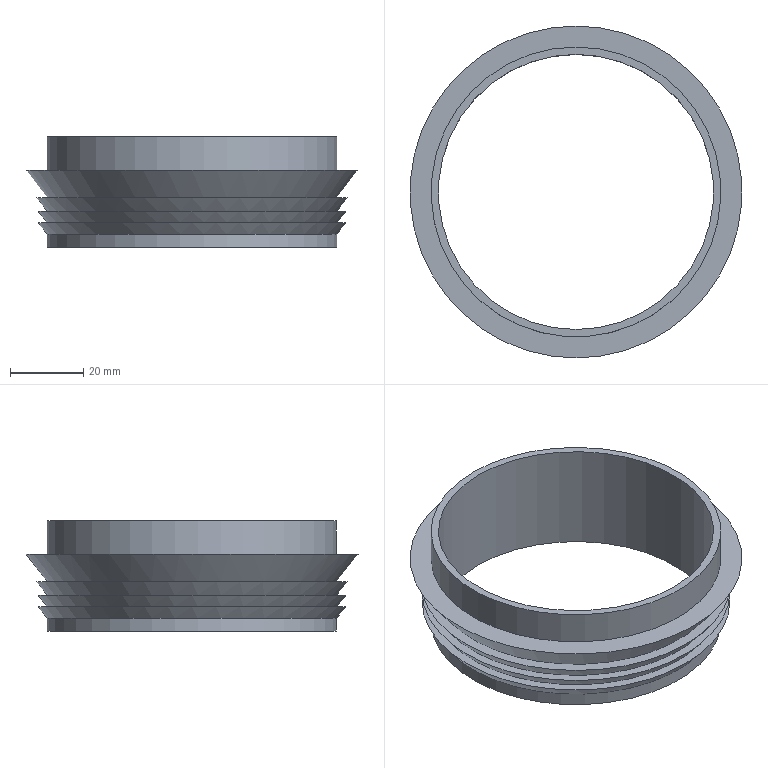Component | NX | CA6140-ZHUZHOU-MIFENGQUAN | 1 solid | 13 faces | box 90.5 x 90.5 x 30 mm | volume 23347 mm3 | plane 6 | cone 4 | cylinder 3 | commonest cylinder face diameters 79 x2 75 x1
STEP:
#1=CARTESIAN_POINT('',(0.,0.,0.));
#2=DIRECTION('',(0.,0.,1.));
#3=DIRECTION('',(1.,0.,0.));
#4=AXIS2_PLACEMENT_3D('',#1,#2,#3);
#5=CARTESIAN_POINT('',(-0.,39.5,-629.951));
#6=VERTEX_POINT('',#5);
#7=CARTESIAN_POINT('',(-0.,0.,-629.951));
#8=DIRECTION('',(0.,0.,-1.));
#9=DIRECTION('',(0.,1.,0.));
#10=AXIS2_PLACEMENT_3D('',#7,#8,#9);
#11=CIRCLE('',#10,39.5);
#12=CARTESIAN_POINT('',(-0.,0.,-629.951));
#13=DIRECTION('',(0.,0.,-1.));
#14=DIRECTION('',(0.,1.,0.));
#15=AXIS2_PLACEMENT_3D('',#12,#13,#14);
#16=CYLINDRICAL_SURFACE('',#15,39.5);
#17=CARTESIAN_POINT('',(0.,0.));
#18=DIRECTION('',(1.,0.));
#19=VECTOR('',#18,1.);
#20=LINE('',#17,#19);
#21=(GEOMETRIC_REPRESENTATION_CONTEXT(2)PARAMETRIC_REPRESENTATION_CONTEXT()REPRESENTATION_CONTEXT('',''));
#22=DEFINITIONAL_REPRESENTATION('',(#20),#21);
#23=PCURVE('',#16,#22);
#24=CARTESIAN_POINT('',(-0.,-39.5,-629.951));
#25=DIRECTION('',(0.,0.,1.));
#26=DIRECTION('',(0.,-1.,0.));
#27=AXIS2_PLACEMENT_3D('',#24,#25,#26);
#28=PLANE('',#27);
#29=CARTESIAN_POINT('',(-79.,0.));
#30=CARTESIAN_POINT('',(-79.,68.416));
#31=CARTESIAN_POINT('',(-19.75,34.208));
#32=CARTESIAN_POINT('',(39.5,0.));
#33=CARTESIAN_POINT('',(-19.75,-34.208));
#34=CARTESIAN_POINT('',(-79.,-68.416));
#35=CARTESIAN_POINT('',(-79.,0.));
#36=(BOUNDED_CURVE()B_SPLINE_CURVE(2,(#29,#30,#31,#32,#33,#34,#35),.UNSPECIFIED.,.T.,.F.)B_SPLINE_CURVE_WITH_KNOTS((1,2,2,2,2,1),(-2.094,0.,2.094,4.189,6.283,8.378),.UNSPECIFIED.)CURVE()GEOMETRIC_REPRESENTATION_ITEM()RATIONAL_B_SPLINE_CURVE((1.,0.5,1.,0.5,1.,0.5,1.))REPRESENTATION_ITEM(''));
#37=(GEOMETRIC_REPRESENTATION_CONTEXT(2)PARAMETRIC_REPRESENTATION_CONTEXT()REPRESENTATION_CONTEXT('',''));
#38=DEFINITIONAL_REPRESENTATION('',(#36),#37);
#39=PCURVE('',#28,#38);
#40=SURFACE_CURVE('',#11,(#23,#39),.PCURVE_S1.);
#41=EDGE_CURVE('',#6,#6,#40,.T.);
#42=ORIENTED_EDGE('',*,*,#41,.F.);
#43=CARTESIAN_POINT('',(-0.,39.5,-626.451));
#44=VERTEX_POINT('',#43);
#45=CARTESIAN_POINT('',(-0.,39.5,-626.451));
#46=CARTESIAN_POINT('',(-0.,39.5,-629.951));
#47=B_SPLINE_CURVE_WITH_KNOTS('',1,(#45,#46),.UNSPECIFIED.,.F.,.F.,(2,2),(-3.5,0.),.PIECEWISE_BEZIER_KNOTS.);
#48=CARTESIAN_POINT('',(0.,0.));
#49=DIRECTION('',(0.,1.));
#50=VECTOR('',#49,1.);
#51=LINE('',#48,#50);
#52=(GEOMETRIC_REPRESENTATION_CONTEXT(2)PARAMETRIC_REPRESENTATION_CONTEXT()REPRESENTATION_CONTEXT('',''));
#53=DEFINITIONAL_REPRESENTATION('',(#51),#52);
#54=PCURVE('',#16,#53);
#55=CARTESIAN_POINT('',(6.283,0.));
#56=DIRECTION('',(0.,1.));
#57=VECTOR('',#56,1.);
#58=LINE('',#55,#57);
#59=(GEOMETRIC_REPRESENTATION_CONTEXT(2)PARAMETRIC_REPRESENTATION_CONTEXT()REPRESENTATION_CONTEXT('',''));
#60=DEFINITIONAL_REPRESENTATION('',(#58),#59);
#61=PCURVE('',#16,#60);
#62=SEAM_CURVE('',#47,(#54,#61),.PCURVE_S1.);
#63=EDGE_CURVE('',#44,#6,#62,.T.);
#64=ORIENTED_EDGE('',*,*,#63,.F.);
#65=CARTESIAN_POINT('',(-0.,0.,-626.451));
#66=DIRECTION('',(0.,0.,-1.));
#67=DIRECTION('',(0.,1.,0.));
#68=AXIS2_PLACEMENT_3D('',#65,#66,#67);
#69=CIRCLE('',#68,39.5);
#70=CARTESIAN_POINT('',(0.,-3.5));
#71=DIRECTION('',(1.,0.));
#72=VECTOR('',#71,1.);
#73=LINE('',#70,#72);
#74=(GEOMETRIC_REPRESENTATION_CONTEXT(2)PARAMETRIC_REPRESENTATION_CONTEXT()REPRESENTATION_CONTEXT('',''));
#75=DEFINITIONAL_REPRESENTATION('',(#73),#74);
#76=PCURVE('',#16,#75);
#77=CARTESIAN_POINT('',(-0.,0.,-623.299));
#78=DIRECTION('',(0.,0.,1.));
#79=DIRECTION('',(0.,-1.,0.));
#80=AXIS2_PLACEMENT_3D('',#77,#78,#79);
#81=CONICAL_SURFACE('',#80,41.963,0.6632);
#82=CARTESIAN_POINT('',(9.425,-3.152));
#83=DIRECTION('',(-1.,0.));
#84=VECTOR('',#83,1.);
#85=LINE('',#82,#84);
#86=(GEOMETRIC_REPRESENTATION_CONTEXT(2)PARAMETRIC_REPRESENTATION_CONTEXT()REPRESENTATION_CONTEXT('',''));
#87=DEFINITIONAL_REPRESENTATION('',(#85),#86);
#88=PCURVE('',#81,#87);
#89=SURFACE_CURVE('',#69,(#76,#88),.PCURVE_S1.);
#90=EDGE_CURVE('',#44,#44,#89,.T.);
#91=ORIENTED_EDGE('',*,*,#90,.T.);
#92=ORIENTED_EDGE('',*,*,#63,.T.);
#93=EDGE_LOOP('',(#42,#64,#91,#92));
#94=FACE_BOUND('',#93,.T.);
#95=ADVANCED_FACE('',(#94),#16,.T.);
#96=CARTESIAN_POINT('',(-0.,-37.5,-629.951));
#97=VERTEX_POINT('',#96);
#98=CARTESIAN_POINT('',(-0.,37.5,-629.951));
#99=VERTEX_POINT('',#98);
#100=CARTESIAN_POINT('',(-0.,0.,-629.951));
#101=DIRECTION('',(0.,0.,-1.));
#102=DIRECTION('',(0.,-1.,0.));
#103=AXIS2_PLACEMENT_3D('',#100,#101,#102);
#104=CIRCLE('',#103,37.5);
#105=CARTESIAN_POINT('',(-2.,0.));
#106=CARTESIAN_POINT('',(-2.,-64.952));
#107=CARTESIAN_POINT('',(-58.25,-32.476));
#108=CARTESIAN_POINT('',(-114.5,-0.));
#109=CARTESIAN_POINT('',(-58.25,32.476));
#110=CARTESIAN_POINT('',(-2.,64.952));
#111=CARTESIAN_POINT('',(-2.,0.));
#112=(BOUNDED_CURVE()B_SPLINE_CURVE(2,(#105,#106,#107,#108,#109,#110,#111),.UNSPECIFIED.,.T.,.F.)B_SPLINE_CURVE_WITH_KNOTS((1,2,2,2,2,1),(-2.094,0.,2.094,4.189,6.283,8.378),.UNSPECIFIED.)CURVE()GEOMETRIC_REPRESENTATION_ITEM()RATIONAL_B_SPLINE_CURVE((1.,0.5,1.,0.5,1.,0.5,1.))REPRESENTATION_ITEM(''));
#113=(GEOMETRIC_REPRESENTATION_CONTEXT(2)PARAMETRIC_REPRESENTATION_CONTEXT()REPRESENTATION_CONTEXT('',''));
#114=DEFINITIONAL_REPRESENTATION('',(#112),#113);
#115=PCURVE('',#28,#114);
#116=CARTESIAN_POINT('',(-0.,0.,-629.951));
#117=DIRECTION('',(0.,0.,-1.));
#118=DIRECTION('',(0.,1.,0.));
#119=AXIS2_PLACEMENT_3D('',#116,#117,#118);
#120=CYLINDRICAL_SURFACE('',#119,37.5);
#121=CARTESIAN_POINT('',(3.142,0.));
#122=DIRECTION('',(1.,0.));
#123=VECTOR('',#122,1.);
#124=LINE('',#121,#123);
#125=(GEOMETRIC_REPRESENTATION_CONTEXT(2)PARAMETRIC_REPRESENTATION_CONTEXT()REPRESENTATION_CONTEXT('',''));
#126=DEFINITIONAL_REPRESENTATION('',(#124),#125);
#127=PCURVE('',#120,#126);
#128=SURFACE_CURVE('',#104,(#115,#127),.PCURVE_S1.);
#129=EDGE_CURVE('',#97,#99,#128,.T.);
#130=ORIENTED_EDGE('',*,*,#129,.F.);
#131=CARTESIAN_POINT('',(-0.,0.,-629.951));
#132=DIRECTION('',(0.,0.,-1.));
#133=DIRECTION('',(0.,-1.,0.));
#134=AXIS2_PLACEMENT_3D('',#131,#132,#133);
#135=CIRCLE('',#134,37.5);
#136=CARTESIAN_POINT('',(-2.,0.));
#137=CARTESIAN_POINT('',(-2.,-64.952));
#138=CARTESIAN_POINT('',(-58.25,-32.476));
#139=CARTESIAN_POINT('',(-114.5,-0.));
#140=CARTESIAN_POINT('',(-58.25,32.476));
#141=CARTESIAN_POINT('',(-2.,64.952));
#142=CARTESIAN_POINT('',(-2.,0.));
#143=(BOUNDED_CURVE()B_SPLINE_CURVE(2,(#136,#137,#138,#139,#140,#141,#142),.UNSPECIFIED.,.T.,.F.)B_SPLINE_CURVE_WITH_KNOTS((1,2,2,2,2,1),(-2.094,0.,2.094,4.189,6.283,8.378),.UNSPECIFIED.)CURVE()GEOMETRIC_REPRESENTATION_ITEM()RATIONAL_B_SPLINE_CURVE((1.,0.5,1.,0.5,1.,0.5,1.))REPRESENTATION_ITEM(''));
#144=(GEOMETRIC_REPRESENTATION_CONTEXT(2)PARAMETRIC_REPRESENTATION_CONTEXT()REPRESENTATION_CONTEXT('',''));
#145=DEFINITIONAL_REPRESENTATION('',(#143),#144);
#146=PCURVE('',#28,#145);
#147=CARTESIAN_POINT('',(-3.142,0.));
#148=DIRECTION('',(1.,0.));
#149=VECTOR('',#148,1.);
#150=LINE('',#147,#149);
#151=(GEOMETRIC_REPRESENTATION_CONTEXT(2)PARAMETRIC_REPRESENTATION_CONTEXT()REPRESENTATION_CONTEXT('',''));
#152=DEFINITIONAL_REPRESENTATION('',(#150),#151);
#153=PCURVE('',#120,#152);
#154=SURFACE_CURVE('',#135,(#146,#153),.PCURVE_S1.);
#155=EDGE_CURVE('',#99,#97,#154,.T.);
#156=ORIENTED_EDGE('',*,*,#155,.F.);
#157=EDGE_LOOP('',(#130,#156));
#158=FACE_BOUND('',#157,.T.);
#159=ORIENTED_EDGE('',*,*,#41,.T.);
#160=EDGE_LOOP('',(#159));
#161=FACE_BOUND('',#160,.T.);
#162=ADVANCED_FACE('',(#158,#161),#28,.F.);
#163=CARTESIAN_POINT('',(-0.,37.5,-599.951));
#164=VERTEX_POINT('',#163);
#165=CARTESIAN_POINT('',(-0.,0.,-599.951));
#166=DIRECTION('',(0.,0.,-1.));
#167=DIRECTION('',(0.,1.,0.));
#168=AXIS2_PLACEMENT_3D('',#165,#166,#167);
#169=CIRCLE('',#168,37.5);
#170=CARTESIAN_POINT('',(0.,-30.));
#171=DIRECTION('',(1.,0.));
#172=VECTOR('',#171,1.);
#173=LINE('',#170,#172);
#174=(GEOMETRIC_REPRESENTATION_CONTEXT(2)PARAMETRIC_REPRESENTATION_CONTEXT()REPRESENTATION_CONTEXT('',''));
#175=DEFINITIONAL_REPRESENTATION('',(#173),#174);
#176=PCURVE('',#120,#175);
#177=CARTESIAN_POINT('',(-0.,-35.5,-599.951));
#178=DIRECTION('',(0.,0.,-1.));
#179=DIRECTION('',(0.,1.,0.));
#180=AXIS2_PLACEMENT_3D('',#177,#178,#179);
#181=PLANE('',#180);
#182=CARTESIAN_POINT('',(35.5,0.));
#183=DIRECTION('',(1.,0.));
#184=AXIS2_PLACEMENT_2D('',#182,#183);
#185=CIRCLE('',#184,37.5);
#186=(GEOMETRIC_REPRESENTATION_CONTEXT(2)PARAMETRIC_REPRESENTATION_CONTEXT()REPRESENTATION_CONTEXT('',''));
#187=DEFINITIONAL_REPRESENTATION('',(#185),#186);
#188=PCURVE('',#181,#187);
#189=SURFACE_CURVE('',#169,(#176,#188),.PCURVE_S1.);
#190=EDGE_CURVE('',#164,#164,#189,.T.);
#191=ORIENTED_EDGE('',*,*,#190,.T.);
#192=CARTESIAN_POINT('',(-0.,37.5,-599.951));
#193=CARTESIAN_POINT('',(-0.,37.5,-629.951));
#194=B_SPLINE_CURVE_WITH_KNOTS('',1,(#192,#193),.UNSPECIFIED.,.F.,.F.,(2,2),(-30.,0.),.PIECEWISE_BEZIER_KNOTS.);
#195=CARTESIAN_POINT('',(6.283,0.));
#196=DIRECTION('',(0.,1.));
#197=VECTOR('',#196,1.);
#198=LINE('',#195,#197);
#199=(GEOMETRIC_REPRESENTATION_CONTEXT(2)PARAMETRIC_REPRESENTATION_CONTEXT()REPRESENTATION_CONTEXT('',''));
#200=DEFINITIONAL_REPRESENTATION('',(#198),#199);
#201=PCURVE('',#120,#200);
#202=CARTESIAN_POINT('',(0.,0.));
#203=DIRECTION('',(0.,1.));
#204=VECTOR('',#203,1.);
#205=LINE('',#202,#204);
#206=(GEOMETRIC_REPRESENTATION_CONTEXT(2)PARAMETRIC_REPRESENTATION_CONTEXT()REPRESENTATION_CONTEXT('',''));
#207=DEFINITIONAL_REPRESENTATION('',(#205),#206);
#208=PCURVE('',#120,#207);
#209=SEAM_CURVE('',#194,(#201,#208),.PCURVE_S1.);
#210=EDGE_CURVE('',#164,#99,#209,.T.);
#211=ORIENTED_EDGE('',*,*,#210,.T.);
#212=ORIENTED_EDGE('',*,*,#129,.F.);
#213=ORIENTED_EDGE('',*,*,#155,.F.);
#214=ORIENTED_EDGE('',*,*,#210,.F.);
#215=EDGE_LOOP('',(#191,#211,#212,#213,#214));
#216=FACE_BOUND('',#215,.F.);
#217=ADVANCED_FACE('',(#216),#120,.F.);
#218=CARTESIAN_POINT('',(-0.,39.5,-599.951));
#219=VERTEX_POINT('',#218);
#220=CARTESIAN_POINT('',(-0.,0.,-599.951));
#221=DIRECTION('',(0.,0.,-1.));
#222=DIRECTION('',(0.,1.,0.));
#223=AXIS2_PLACEMENT_3D('',#220,#221,#222);
#224=CIRCLE('',#223,39.5);
#225=CARTESIAN_POINT('',(35.5,0.));
#226=DIRECTION('',(1.,0.));
#227=AXIS2_PLACEMENT_2D('',#225,#226);
#228=CIRCLE('',#227,39.5);
#229=(GEOMETRIC_REPRESENTATION_CONTEXT(2)PARAMETRIC_REPRESENTATION_CONTEXT()REPRESENTATION_CONTEXT('',''));
#230=DEFINITIONAL_REPRESENTATION('',(#228),#229);
#231=PCURVE('',#181,#230);
#232=CARTESIAN_POINT('',(-0.,0.,-629.951));
#233=DIRECTION('',(0.,0.,-1.));
#234=DIRECTION('',(0.,1.,0.));
#235=AXIS2_PLACEMENT_3D('',#232,#233,#234);
#236=CYLINDRICAL_SURFACE('',#235,39.5);
#237=CARTESIAN_POINT('',(0.,-30.));
#238=DIRECTION('',(1.,0.));
#239=VECTOR('',#238,1.);
#240=LINE('',#237,#239);
#241=(GEOMETRIC_REPRESENTATION_CONTEXT(2)PARAMETRIC_REPRESENTATION_CONTEXT()REPRESENTATION_CONTEXT('',''));
#242=DEFINITIONAL_REPRESENTATION('',(#240),#241);
#243=PCURVE('',#236,#242);
#244=SURFACE_CURVE('',#224,(#231,#243),.PCURVE_S1.);
#245=EDGE_CURVE('',#219,#219,#244,.T.);
#246=ORIENTED_EDGE('',*,*,#245,.F.);
#247=EDGE_LOOP('',(#246));
#248=FACE_BOUND('',#247,.T.);
#249=ORIENTED_EDGE('',*,*,#190,.T.);
#250=EDGE_LOOP('',(#249));
#251=FACE_BOUND('',#250,.T.);
#252=ADVANCED_FACE('',(#248,#251),#181,.F.);
#253=CARTESIAN_POINT('',(-0.,39.5,-608.971));
#254=VERTEX_POINT('',#253);
#255=CARTESIAN_POINT('',(-0.,0.,-608.971));
#256=DIRECTION('',(0.,0.,-1.));
#257=DIRECTION('',(0.,1.,0.));
#258=AXIS2_PLACEMENT_3D('',#255,#256,#257);
#259=CIRCLE('',#258,39.5);
#260=CARTESIAN_POINT('',(0.,-20.98));
#261=DIRECTION('',(1.,0.));
#262=VECTOR('',#261,1.);
#263=LINE('',#260,#262);
#264=(GEOMETRIC_REPRESENTATION_CONTEXT(2)PARAMETRIC_REPRESENTATION_CONTEXT()REPRESENTATION_CONTEXT('',''));
#265=DEFINITIONAL_REPRESENTATION('',(#263),#264);
#266=PCURVE('',#236,#265);
#267=CARTESIAN_POINT('',(-0.,-39.5,-608.971));
#268=DIRECTION('',(0.,0.,-1.));
#269=DIRECTION('',(0.,1.,0.));
#270=AXIS2_PLACEMENT_3D('',#267,#268,#269);
#271=PLANE('',#270);
#272=CARTESIAN_POINT('',(39.5,0.));
#273=DIRECTION('',(1.,0.));
#274=AXIS2_PLACEMENT_2D('',#272,#273);
#275=CIRCLE('',#274,39.5);
#276=(GEOMETRIC_REPRESENTATION_CONTEXT(2)PARAMETRIC_REPRESENTATION_CONTEXT()REPRESENTATION_CONTEXT('',''));
#277=DEFINITIONAL_REPRESENTATION('',(#275),#276);
#278=PCURVE('',#271,#277);
#279=SURFACE_CURVE('',#259,(#266,#278),.PCURVE_S1.);
#280=EDGE_CURVE('',#254,#254,#279,.T.);
#281=ORIENTED_EDGE('',*,*,#280,.F.);
#282=CARTESIAN_POINT('',(-0.,39.5,-599.951));
#283=CARTESIAN_POINT('',(-0.,39.5,-608.971));
#284=B_SPLINE_CURVE_WITH_KNOTS('',1,(#282,#283),.UNSPECIFIED.,.F.,.F.,(2,2),(-30.,-20.98),.PIECEWISE_BEZIER_KNOTS.);
#285=CARTESIAN_POINT('',(0.,0.));
#286=DIRECTION('',(0.,1.));
#287=VECTOR('',#286,1.);
#288=LINE('',#285,#287);
#289=(GEOMETRIC_REPRESENTATION_CONTEXT(2)PARAMETRIC_REPRESENTATION_CONTEXT()REPRESENTATION_CONTEXT('',''));
#290=DEFINITIONAL_REPRESENTATION('',(#288),#289);
#291=PCURVE('',#236,#290);
#292=CARTESIAN_POINT('',(6.283,0.));
#293=DIRECTION('',(0.,1.));
#294=VECTOR('',#293,1.);
#295=LINE('',#292,#294);
#296=(GEOMETRIC_REPRESENTATION_CONTEXT(2)PARAMETRIC_REPRESENTATION_CONTEXT()REPRESENTATION_CONTEXT('',''));
#297=DEFINITIONAL_REPRESENTATION('',(#295),#296);
#298=PCURVE('',#236,#297);
#299=SEAM_CURVE('',#284,(#291,#298),.PCURVE_S1.);
#300=EDGE_CURVE('',#219,#254,#299,.T.);
#301=ORIENTED_EDGE('',*,*,#300,.F.);
#302=ORIENTED_EDGE('',*,*,#245,.T.);
#303=ORIENTED_EDGE('',*,*,#300,.T.);
#304=EDGE_LOOP('',(#281,#301,#302,#303));
#305=FACE_BOUND('',#304,.T.);
#306=ADVANCED_FACE('',(#305),#236,.T.);
#307=CARTESIAN_POINT('',(-0.,45.252,-608.971));
#308=VERTEX_POINT('',#307);
#309=CARTESIAN_POINT('',(-0.,0.,-608.971));
#310=DIRECTION('',(0.,0.,-1.));
#311=DIRECTION('',(0.,1.,0.));
#312=AXIS2_PLACEMENT_3D('',#309,#310,#311);
#313=CIRCLE('',#312,45.252);
#314=CARTESIAN_POINT('',(39.5,0.));
#315=DIRECTION('',(1.,0.));
#316=AXIS2_PLACEMENT_2D('',#314,#315);
#317=CIRCLE('',#316,45.252);
#318=(GEOMETRIC_REPRESENTATION_CONTEXT(2)PARAMETRIC_REPRESENTATION_CONTEXT()REPRESENTATION_CONTEXT('',''));
#319=DEFINITIONAL_REPRESENTATION('',(#317),#318);
#320=PCURVE('',#271,#319);
#321=CARTESIAN_POINT('',(-0.,0.,-608.971));
#322=DIRECTION('',(0.,0.,1.));
#323=DIRECTION('',(0.,-1.,0.));
#324=AXIS2_PLACEMENT_3D('',#321,#322,#323);
#325=CONICAL_SURFACE('',#324,45.252,0.6578);
#326=CARTESIAN_POINT('',(9.425,0.));
#327=DIRECTION('',(-1.,0.));
#328=VECTOR('',#327,1.);
#329=LINE('',#326,#328);
#330=(GEOMETRIC_REPRESENTATION_CONTEXT(2)PARAMETRIC_REPRESENTATION_CONTEXT()REPRESENTATION_CONTEXT('',''));
#331=DEFINITIONAL_REPRESENTATION('',(#329),#330);
#332=PCURVE('',#325,#331);
#333=SURFACE_CURVE('',#313,(#320,#332),.PCURVE_S1.);
#334=EDGE_CURVE('',#308,#308,#333,.T.);
#335=ORIENTED_EDGE('',*,*,#334,.F.);
#336=EDGE_LOOP('',(#335));
#337=FACE_BOUND('',#336,.T.);
#338=ORIENTED_EDGE('',*,*,#280,.T.);
#339=EDGE_LOOP('',(#338));
#340=FACE_BOUND('',#339,.T.);
#341=ADVANCED_FACE('',(#337,#340),#271,.F.);
#342=CARTESIAN_POINT('',(-0.,39.402,-616.543));
#343=VERTEX_POINT('',#342);
#344=CARTESIAN_POINT('',(-0.,0.,-616.543));
#345=DIRECTION('',(0.,0.,-1.));
#346=DIRECTION('',(0.,1.,0.));
#347=AXIS2_PLACEMENT_3D('',#344,#345,#346);
#348=CIRCLE('',#347,39.402);
#349=CARTESIAN_POINT('',(9.425,-7.572));
#350=DIRECTION('',(-1.,0.));
#351=VECTOR('',#350,1.);
#352=LINE('',#349,#351);
#353=(GEOMETRIC_REPRESENTATION_CONTEXT(2)PARAMETRIC_REPRESENTATION_CONTEXT()REPRESENTATION_CONTEXT('',''));
#354=DEFINITIONAL_REPRESENTATION('',(#352),#353);
#355=PCURVE('',#325,#354);
#356=CARTESIAN_POINT('',(-0.,-39.402,-616.543));
#357=DIRECTION('',(0.,0.,-1.));
#358=DIRECTION('',(0.,1.,0.));
#359=AXIS2_PLACEMENT_3D('',#356,#357,#358);
#360=PLANE('',#359);
#361=CARTESIAN_POINT('',(39.402,0.));
#362=DIRECTION('',(1.,0.));
#363=AXIS2_PLACEMENT_2D('',#361,#362);
#364=CIRCLE('',#363,39.402);
#365=(GEOMETRIC_REPRESENTATION_CONTEXT(2)PARAMETRIC_REPRESENTATION_CONTEXT()REPRESENTATION_CONTEXT('',''));
#366=DEFINITIONAL_REPRESENTATION('',(#364),#365);
#367=PCURVE('',#360,#366);
#368=SURFACE_CURVE('',#348,(#355,#367),.PCURVE_S1.);
#369=EDGE_CURVE('',#343,#343,#368,.T.);
#370=ORIENTED_EDGE('',*,*,#369,.F.);
#371=CARTESIAN_POINT('',(-0.,39.402,-616.543));
#372=CARTESIAN_POINT('',(-0.,45.252,-608.971));
#373=B_SPLINE_CURVE_WITH_KNOTS('',1,(#371,#372),.UNSPECIFIED.,.F.,.F.,(2,2),(-9.568,0.),.PIECEWISE_BEZIER_KNOTS.);
#374=CARTESIAN_POINT('',(9.425,0.));
#375=DIRECTION('',(0.,1.));
#376=VECTOR('',#375,1.);
#377=LINE('',#374,#376);
#378=(GEOMETRIC_REPRESENTATION_CONTEXT(2)PARAMETRIC_REPRESENTATION_CONTEXT()REPRESENTATION_CONTEXT('',''));
#379=DEFINITIONAL_REPRESENTATION('',(#377),#378);
#380=PCURVE('',#325,#379);
#381=CARTESIAN_POINT('',(3.142,0.));
#382=DIRECTION('',(0.,1.));
#383=VECTOR('',#382,1.);
#384=LINE('',#381,#383);
#385=(GEOMETRIC_REPRESENTATION_CONTEXT(2)PARAMETRIC_REPRESENTATION_CONTEXT()REPRESENTATION_CONTEXT('',''));
#386=DEFINITIONAL_REPRESENTATION('',(#384),#385);
#387=PCURVE('',#325,#386);
#388=SEAM_CURVE('',#373,(#380,#387),.PCURVE_S1.);
#389=EDGE_CURVE('',#343,#308,#388,.T.);
#390=ORIENTED_EDGE('',*,*,#389,.T.);
#391=ORIENTED_EDGE('',*,*,#334,.T.);
#392=ORIENTED_EDGE('',*,*,#389,.F.);
#393=EDGE_LOOP('',(#370,#390,#391,#392));
#394=FACE_BOUND('',#393,.T.);
#395=ADVANCED_FACE('',(#394),#325,.T.);
#396=CARTESIAN_POINT('',(-0.,42.308,-616.543));
#397=VERTEX_POINT('',#396);
#398=CARTESIAN_POINT('',(-0.,0.,-616.543));
#399=DIRECTION('',(0.,0.,-1.));
#400=DIRECTION('',(0.,1.,0.));
#401=AXIS2_PLACEMENT_3D('',#398,#399,#400);
#402=CIRCLE('',#401,42.308);
#403=CARTESIAN_POINT('',(39.402,0.));
#404=DIRECTION('',(1.,0.));
#405=AXIS2_PLACEMENT_2D('',#403,#404);
#406=CIRCLE('',#405,42.308);
#407=(GEOMETRIC_REPRESENTATION_CONTEXT(2)PARAMETRIC_REPRESENTATION_CONTEXT()REPRESENTATION_CONTEXT('',''));
#408=DEFINITIONAL_REPRESENTATION('',(#406),#407);
#409=PCURVE('',#360,#408);
#410=CARTESIAN_POINT('',(-0.,0.,-616.543));
#411=DIRECTION('',(0.,0.,1.));
#412=DIRECTION('',(0.,-1.,0.));
#413=AXIS2_PLACEMENT_3D('',#410,#411,#412);
#414=CONICAL_SURFACE('',#413,42.308,0.6578);
#415=CARTESIAN_POINT('',(9.425,0.));
#416=DIRECTION('',(-1.,0.));
#417=VECTOR('',#416,1.);
#418=LINE('',#415,#417);
#419=(GEOMETRIC_REPRESENTATION_CONTEXT(2)PARAMETRIC_REPRESENTATION_CONTEXT()REPRESENTATION_CONTEXT('',''));
#420=DEFINITIONAL_REPRESENTATION('',(#418),#419);
#421=PCURVE('',#414,#420);
#422=SURFACE_CURVE('',#402,(#409,#421),.PCURVE_S1.);
#423=EDGE_CURVE('',#397,#397,#422,.T.);
#424=ORIENTED_EDGE('',*,*,#423,.F.);
#425=EDGE_LOOP('',(#424));
#426=FACE_BOUND('',#425,.T.);
#427=ORIENTED_EDGE('',*,*,#369,.T.);
#428=EDGE_LOOP('',(#427));
#429=FACE_BOUND('',#428,.T.);
#430=ADVANCED_FACE('',(#426,#429),#360,.F.);
#431=CARTESIAN_POINT('',(-0.,39.523,-620.147));
#432=VERTEX_POINT('',#431);
#433=CARTESIAN_POINT('',(-0.,0.,-620.147));
#434=DIRECTION('',(0.,0.,-1.));
#435=DIRECTION('',(0.,1.,0.));
#436=AXIS2_PLACEMENT_3D('',#433,#434,#435);
#437=CIRCLE('',#436,39.523);
#438=CARTESIAN_POINT('',(9.425,-3.604));
#439=DIRECTION('',(-1.,0.));
#440=VECTOR('',#439,1.);
#441=LINE('',#438,#440);
#442=(GEOMETRIC_REPRESENTATION_CONTEXT(2)PARAMETRIC_REPRESENTATION_CONTEXT()REPRESENTATION_CONTEXT('',''));
#443=DEFINITIONAL_REPRESENTATION('',(#441),#442);
#444=PCURVE('',#414,#443);
#445=CARTESIAN_POINT('',(-0.,-39.523,-620.147));
#446=DIRECTION('',(0.,0.,-1.));
#447=DIRECTION('',(0.,1.,0.));
#448=AXIS2_PLACEMENT_3D('',#445,#446,#447);
#449=PLANE('',#448);
#450=CARTESIAN_POINT('',(39.523,0.));
#451=DIRECTION('',(1.,0.));
#452=AXIS2_PLACEMENT_2D('',#450,#451);
#453=CIRCLE('',#452,39.523);
#454=(GEOMETRIC_REPRESENTATION_CONTEXT(2)PARAMETRIC_REPRESENTATION_CONTEXT()REPRESENTATION_CONTEXT('',''));
#455=DEFINITIONAL_REPRESENTATION('',(#453),#454);
#456=PCURVE('',#449,#455);
#457=SURFACE_CURVE('',#437,(#444,#456),.PCURVE_S1.);
#458=EDGE_CURVE('',#432,#432,#457,.T.);
#459=ORIENTED_EDGE('',*,*,#458,.F.);
#460=CARTESIAN_POINT('',(-0.,39.523,-620.147));
#461=CARTESIAN_POINT('',(-0.,42.308,-616.543));
#462=B_SPLINE_CURVE_WITH_KNOTS('',1,(#460,#461),.UNSPECIFIED.,.F.,.F.,(2,2),(-4.554,0.),.PIECEWISE_BEZIER_KNOTS.);
#463=CARTESIAN_POINT('',(9.425,0.));
#464=DIRECTION('',(0.,1.));
#465=VECTOR('',#464,1.);
#466=LINE('',#463,#465);
#467=(GEOMETRIC_REPRESENTATION_CONTEXT(2)PARAMETRIC_REPRESENTATION_CONTEXT()REPRESENTATION_CONTEXT('',''));
#468=DEFINITIONAL_REPRESENTATION('',(#466),#467);
#469=PCURVE('',#414,#468);
#470=CARTESIAN_POINT('',(3.142,0.));
#471=DIRECTION('',(0.,1.));
#472=VECTOR('',#471,1.);
#473=LINE('',#470,#472);
#474=(GEOMETRIC_REPRESENTATION_CONTEXT(2)PARAMETRIC_REPRESENTATION_CONTEXT()REPRESENTATION_CONTEXT('',''));
#475=DEFINITIONAL_REPRESENTATION('',(#473),#474);
#476=PCURVE('',#414,#475);
#477=SEAM_CURVE('',#462,(#469,#476),.PCURVE_S1.);
#478=EDGE_CURVE('',#432,#397,#477,.T.);
#479=ORIENTED_EDGE('',*,*,#478,.T.);
#480=ORIENTED_EDGE('',*,*,#423,.T.);
#481=ORIENTED_EDGE('',*,*,#478,.F.);
#482=EDGE_LOOP('',(#459,#479,#480,#481));
#483=FACE_BOUND('',#482,.T.);
#484=ADVANCED_FACE('',(#483),#414,.T.);
#485=CARTESIAN_POINT('',(-0.,41.963,-620.147));
#486=VERTEX_POINT('',#485);
#487=CARTESIAN_POINT('',(-0.,0.,-620.147));
#488=DIRECTION('',(0.,0.,-1.));
#489=DIRECTION('',(0.,1.,0.));
#490=AXIS2_PLACEMENT_3D('',#487,#488,#489);
#491=CIRCLE('',#490,41.963);
#492=CARTESIAN_POINT('',(39.523,0.));
#493=DIRECTION('',(1.,0.));
#494=AXIS2_PLACEMENT_2D('',#492,#493);
#495=CIRCLE('',#494,41.963);
#496=(GEOMETRIC_REPRESENTATION_CONTEXT(2)PARAMETRIC_REPRESENTATION_CONTEXT()REPRESENTATION_CONTEXT('',''));
#497=DEFINITIONAL_REPRESENTATION('',(#495),#496);
#498=PCURVE('',#449,#497);
#499=CARTESIAN_POINT('',(-0.,0.,-620.147));
#500=DIRECTION('',(0.,0.,1.));
#501=DIRECTION('',(0.,-1.,0.));
#502=AXIS2_PLACEMENT_3D('',#499,#500,#501);
#503=CONICAL_SURFACE('',#502,41.963,0.6632);
#504=CARTESIAN_POINT('',(9.425,0.));
#505=DIRECTION('',(-1.,0.));
#506=VECTOR('',#505,1.);
#507=LINE('',#504,#506);
#508=(GEOMETRIC_REPRESENTATION_CONTEXT(2)PARAMETRIC_REPRESENTATION_CONTEXT()REPRESENTATION_CONTEXT('',''));
#509=DEFINITIONAL_REPRESENTATION('',(#507),#508);
#510=PCURVE('',#503,#509);
#511=SURFACE_CURVE('',#491,(#498,#510),.PCURVE_S1.);
#512=EDGE_CURVE('',#486,#486,#511,.T.);
#513=ORIENTED_EDGE('',*,*,#512,.F.);
#514=EDGE_LOOP('',(#513));
#515=FACE_BOUND('',#514,.T.);
#516=ORIENTED_EDGE('',*,*,#458,.T.);
#517=EDGE_LOOP('',(#516));
#518=FACE_BOUND('',#517,.T.);
#519=ADVANCED_FACE('',(#515,#518),#449,.F.);
#520=CARTESIAN_POINT('',(-0.,39.5,-623.299));
#521=VERTEX_POINT('',#520);
#522=CARTESIAN_POINT('',(-0.,0.,-623.299));
#523=DIRECTION('',(0.,0.,-1.));
#524=DIRECTION('',(0.,1.,0.));
#525=AXIS2_PLACEMENT_3D('',#522,#523,#524);
#526=CIRCLE('',#525,39.5);
#527=CARTESIAN_POINT('',(9.425,-3.152));
#528=DIRECTION('',(-1.,0.));
#529=VECTOR('',#528,1.);
#530=LINE('',#527,#529);
#531=(GEOMETRIC_REPRESENTATION_CONTEXT(2)PARAMETRIC_REPRESENTATION_CONTEXT()REPRESENTATION_CONTEXT('',''));
#532=DEFINITIONAL_REPRESENTATION('',(#530),#531);
#533=PCURVE('',#503,#532);
#534=CARTESIAN_POINT('',(-0.,-39.5,-623.299));
#535=DIRECTION('',(0.,0.,-1.));
#536=DIRECTION('',(0.,1.,0.));
#537=AXIS2_PLACEMENT_3D('',#534,#535,#536);
#538=PLANE('',#537);
#539=CARTESIAN_POINT('',(39.5,0.));
#540=DIRECTION('',(1.,0.));
#541=AXIS2_PLACEMENT_2D('',#539,#540);
#542=CIRCLE('',#541,39.5);
#543=(GEOMETRIC_REPRESENTATION_CONTEXT(2)PARAMETRIC_REPRESENTATION_CONTEXT()REPRESENTATION_CONTEXT('',''));
#544=DEFINITIONAL_REPRESENTATION('',(#542),#543);
#545=PCURVE('',#538,#544);
#546=SURFACE_CURVE('',#526,(#533,#545),.PCURVE_S1.);
#547=EDGE_CURVE('',#521,#521,#546,.T.);
#548=ORIENTED_EDGE('',*,*,#547,.F.);
#549=CARTESIAN_POINT('',(-0.,39.5,-623.299));
#550=CARTESIAN_POINT('',(-0.,41.963,-620.147));
#551=B_SPLINE_CURVE_WITH_KNOTS('',1,(#549,#550),.UNSPECIFIED.,.F.,.F.,(2,2),(-4.,0.),.PIECEWISE_BEZIER_KNOTS.);
#552=CARTESIAN_POINT('',(9.425,0.));
#553=DIRECTION('',(0.,1.));
#554=VECTOR('',#553,1.);
#555=LINE('',#552,#554);
#556=(GEOMETRIC_REPRESENTATION_CONTEXT(2)PARAMETRIC_REPRESENTATION_CONTEXT()REPRESENTATION_CONTEXT('',''));
#557=DEFINITIONAL_REPRESENTATION('',(#555),#556);
#558=PCURVE('',#503,#557);
#559=CARTESIAN_POINT('',(3.142,0.));
#560=DIRECTION('',(0.,1.));
#561=VECTOR('',#560,1.);
#562=LINE('',#559,#561);
#563=(GEOMETRIC_REPRESENTATION_CONTEXT(2)PARAMETRIC_REPRESENTATION_CONTEXT()REPRESENTATION_CONTEXT('',''));
#564=DEFINITIONAL_REPRESENTATION('',(#562),#563);
#565=PCURVE('',#503,#564);
#566=SEAM_CURVE('',#551,(#558,#565),.PCURVE_S1.);
#567=EDGE_CURVE('',#521,#486,#566,.T.);
#568=ORIENTED_EDGE('',*,*,#567,.T.);
#569=ORIENTED_EDGE('',*,*,#512,.T.);
#570=ORIENTED_EDGE('',*,*,#567,.F.);
#571=EDGE_LOOP('',(#548,#568,#569,#570));
#572=FACE_BOUND('',#571,.T.);
#573=ADVANCED_FACE('',(#572),#503,.T.);
#574=CARTESIAN_POINT('',(-0.,41.963,-623.299));
#575=VERTEX_POINT('',#574);
#576=CARTESIAN_POINT('',(-0.,0.,-623.299));
#577=DIRECTION('',(0.,0.,-1.));
#578=DIRECTION('',(0.,1.,0.));
#579=AXIS2_PLACEMENT_3D('',#576,#577,#578);
#580=CIRCLE('',#579,41.963);
#581=CARTESIAN_POINT('',(39.5,0.));
#582=DIRECTION('',(1.,0.));
#583=AXIS2_PLACEMENT_2D('',#581,#582);
#584=CIRCLE('',#583,41.963);
#585=(GEOMETRIC_REPRESENTATION_CONTEXT(2)PARAMETRIC_REPRESENTATION_CONTEXT()REPRESENTATION_CONTEXT('',''));
#586=DEFINITIONAL_REPRESENTATION('',(#584),#585);
#587=PCURVE('',#538,#586);
#588=CARTESIAN_POINT('',(9.425,0.));
#589=DIRECTION('',(-1.,0.));
#590=VECTOR('',#589,1.);
#591=LINE('',#588,#590);
#592=(GEOMETRIC_REPRESENTATION_CONTEXT(2)PARAMETRIC_REPRESENTATION_CONTEXT()REPRESENTATION_CONTEXT('',''));
#593=DEFINITIONAL_REPRESENTATION('',(#591),#592);
#594=PCURVE('',#81,#593);
#595=SURFACE_CURVE('',#580,(#587,#594),.PCURVE_S1.);
#596=EDGE_CURVE('',#575,#575,#595,.T.);
#597=ORIENTED_EDGE('',*,*,#596,.F.);
#598=EDGE_LOOP('',(#597));
#599=FACE_BOUND('',#598,.T.);
#600=ORIENTED_EDGE('',*,*,#547,.T.);
#601=EDGE_LOOP('',(#600));
#602=FACE_BOUND('',#601,.T.);
#603=ADVANCED_FACE('',(#599,#602),#538,.F.);
#604=ORIENTED_EDGE('',*,*,#90,.F.);
#605=CARTESIAN_POINT('',(-0.,39.5,-626.451));
#606=CARTESIAN_POINT('',(-0.,41.963,-623.299));
#607=B_SPLINE_CURVE_WITH_KNOTS('',1,(#605,#606),.UNSPECIFIED.,.F.,.F.,(2,2),(-4.,0.),.PIECEWISE_BEZIER_KNOTS.);
#608=CARTESIAN_POINT('',(9.425,0.));
#609=DIRECTION('',(0.,1.));
#610=VECTOR('',#609,1.);
#611=LINE('',#608,#610);
#612=(GEOMETRIC_REPRESENTATION_CONTEXT(2)PARAMETRIC_REPRESENTATION_CONTEXT()REPRESENTATION_CONTEXT('',''));
#613=DEFINITIONAL_REPRESENTATION('',(#611),#612);
#614=PCURVE('',#81,#613);
#615=CARTESIAN_POINT('',(3.142,0.));
#616=DIRECTION('',(0.,1.));
#617=VECTOR('',#616,1.);
#618=LINE('',#615,#617);
#619=(GEOMETRIC_REPRESENTATION_CONTEXT(2)PARAMETRIC_REPRESENTATION_CONTEXT()REPRESENTATION_CONTEXT('',''));
#620=DEFINITIONAL_REPRESENTATION('',(#618),#619);
#621=PCURVE('',#81,#620);
#622=SEAM_CURVE('',#607,(#614,#621),.PCURVE_S1.);
#623=EDGE_CURVE('',#44,#575,#622,.T.);
#624=ORIENTED_EDGE('',*,*,#623,.T.);
#625=ORIENTED_EDGE('',*,*,#596,.T.);
#626=ORIENTED_EDGE('',*,*,#623,.F.);
#627=EDGE_LOOP('',(#604,#624,#625,#626));
#628=FACE_BOUND('',#627,.T.);
#629=ADVANCED_FACE('',(#628),#81,.T.);
#630=CLOSED_SHELL('',(#95,#162,#217,#252,#306,#341,#395,#430,#484,#519,#573,#603,#629));
#631=MANIFOLD_SOLID_BREP('',#630);
#632=(LENGTH_UNIT()NAMED_UNIT(*)SI_UNIT(.MILLI.,.METRE.));
#633=UNCERTAINTY_MEASURE_WITH_UNIT(LENGTH_MEASURE(0.00001),#632,'','');
#634=(NAMED_UNIT(*)PLANE_ANGLE_UNIT()SI_UNIT($,.RADIAN.));
#635=(NAMED_UNIT(*)SI_UNIT($,.STERADIAN.)SOLID_ANGLE_UNIT());
#636=(GEOMETRIC_REPRESENTATION_CONTEXT(3)GLOBAL_UNCERTAINTY_ASSIGNED_CONTEXT((#633))GLOBAL_UNIT_ASSIGNED_CONTEXT((#632,#634,#635))REPRESENTATION_CONTEXT('',''));
#637=ADVANCED_BREP_SHAPE_REPRESENTATION('',(#4,#631),#636);